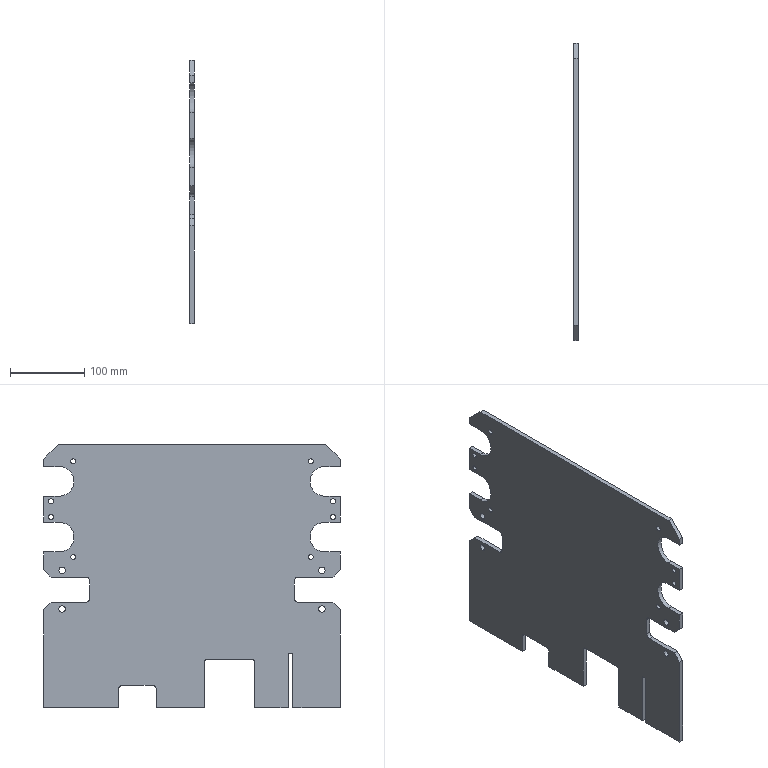Component | SolidWorks | THK-B1002RollerBracketRight-1 | 1 solid | 80 faces | box 6 x 400 x 355 mm | volume 746439 mm3 | plane 44 | cylinder 36 | commonest cylinder face diameters 6.8 x16 9 x8 40 x4 10 x4 8 x4 | material Q235A
build123d program:
from build123d import *

# Parameters (mm, degrees)
BOSS_EXTRUDE1_DEPTH      = 3
CHAMFER1_SIZE            = 10
FILLET1_R                = 5
FILLET2_R                = 4
M8_TAPPED_HOLE1_D        = 6.8
F_9_0_9_DIAMETER_HOLE1_D = 9
CHAMFER2_SIZE            = 20


with BuildPart() as part:
    # Sketch1 → Boss-Extrude1 (new, symmetric)
    with BuildSketch(Plane(origin=(0, 0, 0), x_dir=(0, 0, -1), z_dir=(1, 0, 0))):
        with BuildLine():
            Line((-255, 200), (-113, 200))
            Line((-113, 200), (-113, 138))
            Line((-113, 138), (-79, 138))
            Line((-79, 138), (-79, 200))
            Line((-79, 200), (-45, 200))
            Line((-45, 200), (-45, 179))
            ThreePointArc((-45, 179), (-25, 159), (-5, 179))
            Line((-5, 179), (-5, 200))
            Line((-5, 200), (30, 200))
            Line((30, 200), (30, 179))
            ThreePointArc((30, 179), (50, 159), (70, 179))
            Line((70, 179), (70, 200))
            Line((70, 200), (100, 200))
            Line((100, 200), (100, -200))
            Line((100, -200), (70, -200))
            Line((70, -200), (70, -179))
            ThreePointArc((70, -179), (50, -159), (30, -179))
            Line((30, -179), (30, -200))
            Line((30, -200), (-5, -200))
            Line((-5, -200), (-5, -179))
            ThreePointArc((-5, -179), (-25, -159), (-45, -179))
            Line((-45, -179), (-45, -200))
            Line((-45, -200), (-79, -200))
            Line((-79, -200), (-79, -138))
            Line((-79, -138), (-113, -138))
            Line((-113, -138), (-113, -200))
            Line((-113, -200), (-255, -200))
            Line((-255, -200), (-255, -136))
            Line((-255, -136), (-182, -136))
            Line((-182, -136), (-182, -129.5))
            Line((-182, -129.5), (-255, -129.5))
            Line((-255, -129.5), (-255, -84.5))
            Line((-255, -84.5), (-190, -84.5))
            Line((-190, -84.5), (-190, -16.5))
            Line((-190, -16.5), (-255, -16.5))
            Line((-255, -16.5), (-255, 48.5))
            Line((-255, 48.5), (-225, 48.5))
            Line((-225, 48.5), (-225, 98.5))
            Line((-225, 98.5), (-255, 98.5))
            Line((-255, 98.5), (-255, 200))
        make_face()
    extrude(amount=BOSS_EXTRUDE1_DEPTH, both=True)

    # Chamfer1
    chamfer1_edges = [part.edges().sort_by_distance(p)[0] for p in [
        (0, 200, 113),
        (0, 200, 79),
        (0, -200, 79),
        (0, -200, 113),
    ]]
    chamfer(chamfer1_edges, length=CHAMFER1_SIZE)

    # Fillet1
    fillet1_edges = [part.edges().sort_by_distance(p)[0] for p in [
        (0, 138, 113),
        (0, 138, 79),
        (0, -138, 79),
        (0, -138, 113),
    ]]
    fillet(fillet1_edges, radius=FILLET1_R)

    # Fillet2
    fillet2_edges = [part.edges().sort_by_distance(p)[0] for p in [
        (0, -84.5, 190),
        (0, -16.5, 190),
        (0, 48.5, 225),
        (0, 98.5, 225),
    ]]
    fillet(fillet2_edges, radius=FILLET2_R)

    # M8 Tapped Hole1 (through all)
    with Locations(Plane(origin=(3, 0, 0), x_dir=(0, 0, -1), z_dir=(1, 0, 0))):
        with Locations((2, 190), (23, 190), (-52, 160), (77, 160), (77, -160), (23, -190), (2, -190), (-52, -160)):
            Hole(M8_TAPPED_HOLE1_D / 2)

    # 9.0 _9_ Diameter Hole1 (through all)
    with Locations(Plane(origin=(3, 0, 0), x_dir=(0, 0, -1), z_dir=(1, 0, 0))):
        with Locations((-122, 175), (-70, 175), (-70, -175), (-122, -175)):
            Hole(F_9_0_9_DIAMETER_HOLE1_D / 2)

    # Chamfer2
    chamfer2_edges = [part.edges().sort_by_distance(p)[0] for p in [
        (0, 200, -100),
        (0, -200, -100),
    ]]
    chamfer(chamfer2_edges, length=CHAMFER2_SIZE)


solid = part.part

# Placed as in the assembly
solid = solid.moved(Location((130, 0, 0), (-180, 0, 180)))